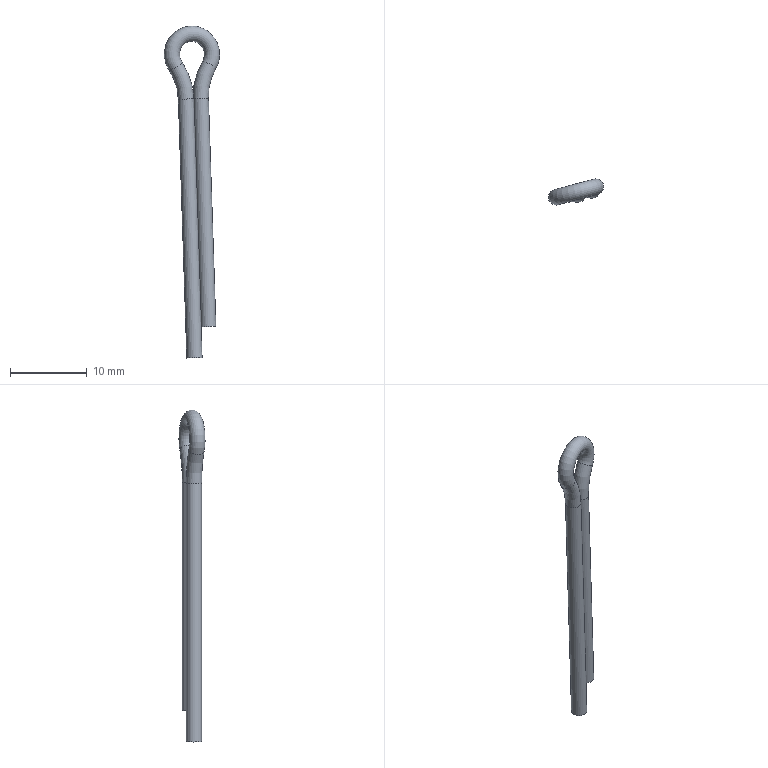Component | NX | 1 | 1 solid | 7 faces | box 7.22 x 3.4 x 43.24 mm | volume 264 mm3 | torus 3 | cylinder 2 | plane 2 | commonest cylinder face diameters 2 x2
STEP:
#1=CARTESIAN_POINT('',(0.,0.,0.));
#2=DIRECTION('',(0.,0.,1.));
#3=DIRECTION('',(1.,0.,0.));
#4=AXIS2_PLACEMENT_3D('',#1,#2,#3);
#5=CARTESIAN_POINT('',(-221.029,-44.318,113.398));
#6=VERTEX_POINT('',#5);
#7=CARTESIAN_POINT('',(-221.287,-43.352,113.39));
#8=DIRECTION('',(0.03267,-0.,-0.9995));
#9=DIRECTION('',(0.2584,-0.966,0.008448));
#10=AXIS2_PLACEMENT_3D('',#7,#8,#9);
#11=CIRCLE('',#10,1.);
#12=CARTESIAN_POINT('',(-221.287,-43.352,113.39));
#13=DIRECTION('',(0.03267,0.,-0.9995));
#14=DIRECTION('',(-0.2584,0.966,-0.008448));
#15=AXIS2_PLACEMENT_3D('',#12,#13,#14);
#16=CYLINDRICAL_SURFACE('',#15,1.);
#17=CARTESIAN_POINT('',(3.142,-0.));
#18=DIRECTION('',(1.,0.));
#19=VECTOR('',#18,1.);
#20=LINE('',#17,#19);
#21=(GEOMETRIC_REPRESENTATION_CONTEXT(2)PARAMETRIC_REPRESENTATION_CONTEXT()REPRESENTATION_CONTEXT('',''));
#22=DEFINITIONAL_REPRESENTATION('',(#20),#21);
#23=PCURVE('',#16,#22);
#24=CARTESIAN_POINT('',(-213.563,-41.284,113.642));
#25=DIRECTION('',(0.2584,-0.966,0.008448));
#26=DIRECTION('',(0.03267,-0.,-0.9995));
#27=AXIS2_PLACEMENT_3D('',#24,#25,#26);
#28=TOROIDAL_SURFACE('',#27,8.,1.);
#29=CARTESIAN_POINT('',(4.712,7.854));
#30=DIRECTION('',(0.,-1.));
#31=VECTOR('',#30,1.);
#32=LINE('',#29,#31);
#33=(GEOMETRIC_REPRESENTATION_CONTEXT(2)PARAMETRIC_REPRESENTATION_CONTEXT()REPRESENTATION_CONTEXT('',''));
#34=DEFINITIONAL_REPRESENTATION('',(#32),#33);
#35=PCURVE('',#28,#34);
#36=SURFACE_CURVE('',#11,(#23,#35),.PCURVE_S1.);
#37=EDGE_CURVE('',#6,#6,#36,.T.);
#38=ORIENTED_EDGE('',*,*,#37,.T.);
#39=CARTESIAN_POINT('',(-220.058,-44.318,83.701));
#40=VERTEX_POINT('',#39);
#41=CARTESIAN_POINT('',(-221.029,-44.318,113.398));
#42=CARTESIAN_POINT('',(-220.058,-44.318,83.701));
#43=B_SPLINE_CURVE_WITH_KNOTS('',1,(#41,#42),.UNSPECIFIED.,.F.,.F.,(2,2),(-0.,29.713),.PIECEWISE_BEZIER_KNOTS.);
#44=CARTESIAN_POINT('',(9.425,0.));
#45=DIRECTION('',(0.,1.));
#46=VECTOR('',#45,1.);
#47=LINE('',#44,#46);
#48=(GEOMETRIC_REPRESENTATION_CONTEXT(2)PARAMETRIC_REPRESENTATION_CONTEXT()REPRESENTATION_CONTEXT('',''));
#49=DEFINITIONAL_REPRESENTATION('',(#47),#48);
#50=PCURVE('',#16,#49);
#51=CARTESIAN_POINT('',(3.142,0.));
#52=DIRECTION('',(0.,1.));
#53=VECTOR('',#52,1.);
#54=LINE('',#51,#53);
#55=(GEOMETRIC_REPRESENTATION_CONTEXT(2)PARAMETRIC_REPRESENTATION_CONTEXT()REPRESENTATION_CONTEXT('',''));
#56=DEFINITIONAL_REPRESENTATION('',(#54),#55);
#57=PCURVE('',#16,#56);
#58=SEAM_CURVE('',#43,(#50,#57),.PCURVE_S1.);
#59=EDGE_CURVE('',#6,#40,#58,.T.);
#60=ORIENTED_EDGE('',*,*,#59,.T.);
#61=CARTESIAN_POINT('',(-220.316,-43.352,83.693));
#62=DIRECTION('',(0.03267,-0.,-0.9995));
#63=DIRECTION('',(0.2584,-0.966,0.008448));
#64=AXIS2_PLACEMENT_3D('',#61,#62,#63);
#65=CIRCLE('',#64,1.);
#66=CARTESIAN_POINT('',(3.142,29.713));
#67=DIRECTION('',(1.,0.));
#68=VECTOR('',#67,1.);
#69=LINE('',#66,#68);
#70=(GEOMETRIC_REPRESENTATION_CONTEXT(2)PARAMETRIC_REPRESENTATION_CONTEXT()REPRESENTATION_CONTEXT('',''));
#71=DEFINITIONAL_REPRESENTATION('',(#69),#70);
#72=PCURVE('',#16,#71);
#73=CARTESIAN_POINT('',(-220.316,-43.352,83.693));
#74=DIRECTION('',(0.03267,-0.,-0.9995));
#75=DIRECTION('',(0.2584,-0.966,0.008448));
#76=AXIS2_PLACEMENT_3D('',#73,#74,#75);
#77=PLANE('',#76);
#78=CARTESIAN_POINT('',(0.,0.));
#79=DIRECTION('',(1.,0.));
#80=AXIS2_PLACEMENT_2D('',#78,#79);
#81=CIRCLE('',#80,1.);
#82=(GEOMETRIC_REPRESENTATION_CONTEXT(2)PARAMETRIC_REPRESENTATION_CONTEXT()REPRESENTATION_CONTEXT('',''));
#83=DEFINITIONAL_REPRESENTATION('',(#81),#82);
#84=PCURVE('',#77,#83);
#85=SURFACE_CURVE('',#65,(#72,#84),.PCURVE_S1.);
#86=EDGE_CURVE('',#40,#40,#85,.T.);
#87=ORIENTED_EDGE('',*,*,#86,.F.);
#88=ORIENTED_EDGE('',*,*,#59,.F.);
#89=EDGE_LOOP('',(#38,#60,#87,#88));
#90=FACE_BOUND('',#89,.T.);
#91=ADVANCED_FACE('',(#90),#16,.T.);
#92=CARTESIAN_POINT('',(-219.943,-43.99,117.763));
#93=VERTEX_POINT('',#92);
#94=CARTESIAN_POINT('',(-220.201,-43.024,117.754));
#95=DIRECTION('',(-0.4947,-0.1398,-0.8577));
#96=DIRECTION('',(0.2584,-0.966,0.008448));
#97=AXIS2_PLACEMENT_3D('',#94,#95,#96);
#98=CIRCLE('',#97,1.);
#99=CARTESIAN_POINT('',(4.141,7.854));
#100=DIRECTION('',(0.,-1.));
#101=VECTOR('',#100,1.);
#102=LINE('',#99,#101);
#103=(GEOMETRIC_REPRESENTATION_CONTEXT(2)PARAMETRIC_REPRESENTATION_CONTEXT()REPRESENTATION_CONTEXT('',''));
#104=DEFINITIONAL_REPRESENTATION('',(#102),#103);
#105=PCURVE('',#28,#104);
#106=CARTESIAN_POINT('',(-222.442,-43.611,119.142));
#107=DIRECTION('',(-0.2584,0.966,-0.008448));
#108=DIRECTION('',(-0.03267,0.,0.9995));
#109=AXIS2_PLACEMENT_3D('',#106,#107,#108);
#110=TOROIDAL_SURFACE('',#109,2.7,1.);
#111=CARTESIAN_POINT('',(8.425,10.996));
#112=DIRECTION('',(0.,-1.));
#113=VECTOR('',#112,1.);
#114=LINE('',#111,#113);
#115=(GEOMETRIC_REPRESENTATION_CONTEXT(2)PARAMETRIC_REPRESENTATION_CONTEXT()REPRESENTATION_CONTEXT('',''));
#116=DEFINITIONAL_REPRESENTATION('',(#114),#115);
#117=PCURVE('',#110,#116);
#118=SURFACE_CURVE('',#98,(#105,#117),.PCURVE_S1.);
#119=EDGE_CURVE('',#93,#93,#118,.T.);
#120=ORIENTED_EDGE('',*,*,#119,.T.);
#121=CARTESIAN_POINT('',(-219.943,-43.99,117.763));
#122=CARTESIAN_POINT('',(-220.321,-44.097,117.108));
#123=CARTESIAN_POINT('',(-220.625,-44.184,116.409));
#124=CARTESIAN_POINT('',(-220.851,-44.251,115.679));
#125=CARTESIAN_POINT('',(-220.994,-44.296,114.926));
#126=CARTESIAN_POINT('',(-221.054,-44.318,114.162));
#127=CARTESIAN_POINT('',(-221.029,-44.318,113.398));
#128=(BOUNDED_CURVE()B_SPLINE_CURVE(6,(#121,#122,#123,#124,#125,#126,#127),.UNSPECIFIED.,.F.,.F.)B_SPLINE_CURVE_WITH_KNOTS((7,7),(4.141,4.712),.PIECEWISE_BEZIER_KNOTS.)CURVE()GEOMETRIC_REPRESENTATION_ITEM()RATIONAL_B_SPLINE_CURVE((1.004,1.001,0.9997,0.9992,0.9997,1.001,1.004))REPRESENTATION_ITEM(''));
#129=CARTESIAN_POINT('',(0.,1.571));
#130=DIRECTION('',(1.,0.));
#131=VECTOR('',#130,1.);
#132=LINE('',#129,#131);
#133=(GEOMETRIC_REPRESENTATION_CONTEXT(2)PARAMETRIC_REPRESENTATION_CONTEXT()REPRESENTATION_CONTEXT('',''));
#134=DEFINITIONAL_REPRESENTATION('',(#132),#133);
#135=PCURVE('',#28,#134);
#136=CARTESIAN_POINT('',(0.,7.854));
#137=DIRECTION('',(1.,0.));
#138=VECTOR('',#137,1.);
#139=LINE('',#136,#138);
#140=(GEOMETRIC_REPRESENTATION_CONTEXT(2)PARAMETRIC_REPRESENTATION_CONTEXT()REPRESENTATION_CONTEXT('',''));
#141=DEFINITIONAL_REPRESENTATION('',(#139),#140);
#142=PCURVE('',#28,#141);
#143=SEAM_CURVE('',#128,(#135,#142),.PCURVE_S1.);
#144=EDGE_CURVE('',#93,#6,#143,.T.);
#145=ORIENTED_EDGE('',*,*,#144,.T.);
#146=ORIENTED_EDGE('',*,*,#37,.F.);
#147=ORIENTED_EDGE('',*,*,#144,.F.);
#148=EDGE_LOOP('',(#120,#145,#146,#147));
#149=FACE_BOUND('',#148,.T.);
#150=ADVANCED_FACE('',(#149),#28,.T.);
#151=CARTESIAN_POINT('',(-224.328,-45.164,117.62));
#152=VERTEX_POINT('',#151);
#153=CARTESIAN_POINT('',(-224.587,-44.198,117.611));
#154=DIRECTION('',(-0.5497,-0.1398,0.8236));
#155=DIRECTION('',(0.2584,-0.966,0.008448));
#156=AXIS2_PLACEMENT_3D('',#153,#154,#155);
#157=CIRCLE('',#156,1.);
#158=CARTESIAN_POINT('',(4.141,10.996));
#159=DIRECTION('',(0.,-1.));
#160=VECTOR('',#159,1.);
#161=LINE('',#158,#160);
#162=(GEOMETRIC_REPRESENTATION_CONTEXT(2)PARAMETRIC_REPRESENTATION_CONTEXT()REPRESENTATION_CONTEXT('',''));
#163=DEFINITIONAL_REPRESENTATION('',(#161),#162);
#164=PCURVE('',#110,#163);
#165=CARTESIAN_POINT('',(-230.942,-45.938,113.074));
#166=DIRECTION('',(0.2584,-0.966,0.008448));
#167=DIRECTION('',(0.03267,-0.,-0.9995));
#168=AXIS2_PLACEMENT_3D('',#165,#166,#167);
#169=TOROIDAL_SURFACE('',#168,8.,1.);
#170=CARTESIAN_POINT('',(8.425,7.854));
#171=DIRECTION('',(0.,-1.));
#172=VECTOR('',#171,1.);
#173=LINE('',#170,#172);
#174=(GEOMETRIC_REPRESENTATION_CONTEXT(2)PARAMETRIC_REPRESENTATION_CONTEXT()REPRESENTATION_CONTEXT('',''));
#175=DEFINITIONAL_REPRESENTATION('',(#173),#174);
#176=PCURVE('',#169,#175);
#177=SURFACE_CURVE('',#157,(#164,#176),.PCURVE_S1.);
#178=EDGE_CURVE('',#152,#152,#177,.T.);
#179=ORIENTED_EDGE('',*,*,#178,.T.);
#180=CARTESIAN_POINT('',(-224.328,-45.164,117.62));
#181=CARTESIAN_POINT('',(-225.035,-45.344,118.678));
#182=CARTESIAN_POINT('',(-225.194,-45.374,120.127));
#183=CARTESIAN_POINT('',(-224.575,-45.195,121.618));
#184=CARTESIAN_POINT('',(-223.187,-44.815,122.641));
#185=CARTESIAN_POINT('',(-221.41,-44.339,122.699));
#186=CARTESIAN_POINT('',(-219.958,-43.959,121.769));
#187=CARTESIAN_POINT('',(-219.242,-43.78,120.322));
#188=CARTESIAN_POINT('',(-219.307,-43.81,118.865));
#189=CARTESIAN_POINT('',(-219.943,-43.99,117.763));
#190=B_SPLINE_CURVE_WITH_KNOTS('',9,(#180,#181,#182,#183,#184,#185,#186,#187,#188,#189),.UNSPECIFIED.,.F.,.F.,(10,10),(4.141,8.425),.PIECEWISE_BEZIER_KNOTS.);
#191=CARTESIAN_POINT('',(0.,4.712));
#192=DIRECTION('',(1.,0.));
#193=VECTOR('',#192,1.);
#194=LINE('',#191,#193);
#195=(GEOMETRIC_REPRESENTATION_CONTEXT(2)PARAMETRIC_REPRESENTATION_CONTEXT()REPRESENTATION_CONTEXT('',''));
#196=DEFINITIONAL_REPRESENTATION('',(#194),#195);
#197=PCURVE('',#110,#196);
#198=CARTESIAN_POINT('',(0.,10.996));
#199=DIRECTION('',(1.,0.));
#200=VECTOR('',#199,1.);
#201=LINE('',#198,#200);
#202=(GEOMETRIC_REPRESENTATION_CONTEXT(2)PARAMETRIC_REPRESENTATION_CONTEXT()REPRESENTATION_CONTEXT('',''));
#203=DEFINITIONAL_REPRESENTATION('',(#201),#202);
#204=PCURVE('',#110,#203);
#205=SEAM_CURVE('',#190,(#197,#204),.PCURVE_S1.);
#206=EDGE_CURVE('',#152,#93,#205,.T.);
#207=ORIENTED_EDGE('',*,*,#206,.T.);
#208=ORIENTED_EDGE('',*,*,#119,.F.);
#209=ORIENTED_EDGE('',*,*,#206,.F.);
#210=EDGE_LOOP('',(#179,#207,#208,#209));
#211=FACE_BOUND('',#210,.T.);
#212=ADVANCED_FACE('',(#211),#110,.T.);
#213=CARTESIAN_POINT('',(-222.96,-44.836,113.335));
#214=VERTEX_POINT('',#213);
#215=CARTESIAN_POINT('',(-223.218,-43.87,113.327));
#216=DIRECTION('',(-0.03267,0.,0.9995));
#217=DIRECTION('',(0.2584,-0.966,0.008448));
#218=AXIS2_PLACEMENT_3D('',#215,#216,#217);
#219=CIRCLE('',#218,1.);
#220=CARTESIAN_POINT('',(7.854,7.854));
#221=DIRECTION('',(0.,-1.));
#222=VECTOR('',#221,1.);
#223=LINE('',#220,#222);
#224=(GEOMETRIC_REPRESENTATION_CONTEXT(2)PARAMETRIC_REPRESENTATION_CONTEXT()REPRESENTATION_CONTEXT('',''));
#225=DEFINITIONAL_REPRESENTATION('',(#223),#224);
#226=PCURVE('',#169,#225);
#227=CARTESIAN_POINT('',(-223.218,-43.87,113.327));
#228=DIRECTION('',(0.03267,0.,-0.9995));
#229=DIRECTION('',(-0.2584,0.966,-0.008448));
#230=AXIS2_PLACEMENT_3D('',#227,#228,#229);
#231=CYLINDRICAL_SURFACE('',#230,1.);
#232=CARTESIAN_POINT('',(9.425,0.));
#233=DIRECTION('',(-1.,0.));
#234=VECTOR('',#233,1.);
#235=LINE('',#232,#234);
#236=(GEOMETRIC_REPRESENTATION_CONTEXT(2)PARAMETRIC_REPRESENTATION_CONTEXT()REPRESENTATION_CONTEXT('',''));
#237=DEFINITIONAL_REPRESENTATION('',(#235),#236);
#238=PCURVE('',#231,#237);
#239=SURFACE_CURVE('',#219,(#226,#238),.PCURVE_S1.);
#240=EDGE_CURVE('',#214,#214,#239,.T.);
#241=ORIENTED_EDGE('',*,*,#240,.T.);
#242=CARTESIAN_POINT('',(-222.96,-44.836,113.335));
#243=CARTESIAN_POINT('',(-222.985,-44.836,114.099));
#244=CARTESIAN_POINT('',(-223.094,-44.858,114.857));
#245=CARTESIAN_POINT('',(-223.286,-44.903,115.599));
#246=CARTESIAN_POINT('',(-223.559,-44.97,116.314));
#247=CARTESIAN_POINT('',(-223.908,-45.057,116.99));
#248=CARTESIAN_POINT('',(-224.328,-45.164,117.62));
#249=(BOUNDED_CURVE()B_SPLINE_CURVE(6,(#242,#243,#244,#245,#246,#247,#248),.UNSPECIFIED.,.F.,.F.)B_SPLINE_CURVE_WITH_KNOTS((7,7),(1.571,2.142),.PIECEWISE_BEZIER_KNOTS.)CURVE()GEOMETRIC_REPRESENTATION_ITEM()RATIONAL_B_SPLINE_CURVE((1.004,1.001,0.9997,0.9992,0.9997,1.001,1.004))REPRESENTATION_ITEM(''));
#250=CARTESIAN_POINT('',(6.283,1.571));
#251=DIRECTION('',(1.,0.));
#252=VECTOR('',#251,1.);
#253=LINE('',#250,#252);
#254=(GEOMETRIC_REPRESENTATION_CONTEXT(2)PARAMETRIC_REPRESENTATION_CONTEXT()REPRESENTATION_CONTEXT('',''));
#255=DEFINITIONAL_REPRESENTATION('',(#253),#254);
#256=PCURVE('',#169,#255);
#257=CARTESIAN_POINT('',(6.283,7.854));
#258=DIRECTION('',(1.,0.));
#259=VECTOR('',#258,1.);
#260=LINE('',#257,#259);
#261=(GEOMETRIC_REPRESENTATION_CONTEXT(2)PARAMETRIC_REPRESENTATION_CONTEXT()REPRESENTATION_CONTEXT('',''));
#262=DEFINITIONAL_REPRESENTATION('',(#260),#261);
#263=PCURVE('',#169,#262);
#264=SEAM_CURVE('',#249,(#256,#263),.PCURVE_S1.);
#265=EDGE_CURVE('',#214,#152,#264,.T.);
#266=ORIENTED_EDGE('',*,*,#265,.T.);
#267=ORIENTED_EDGE('',*,*,#178,.F.);
#268=ORIENTED_EDGE('',*,*,#265,.F.);
#269=EDGE_LOOP('',(#241,#266,#267,#268));
#270=FACE_BOUND('',#269,.T.);
#271=ADVANCED_FACE('',(#270),#169,.T.);
#272=ORIENTED_EDGE('',*,*,#240,.F.);
#273=CARTESIAN_POINT('',(-221.858,-44.836,79.64));
#274=VERTEX_POINT('',#273);
#275=CARTESIAN_POINT('',(-222.96,-44.836,113.335));
#276=CARTESIAN_POINT('',(-221.858,-44.836,79.64));
#277=B_SPLINE_CURVE_WITH_KNOTS('',1,(#275,#276),.UNSPECIFIED.,.F.,.F.,(2,2),(0.,33.713),.PIECEWISE_BEZIER_KNOTS.);
#278=CARTESIAN_POINT('',(9.425,0.));
#279=DIRECTION('',(0.,1.));
#280=VECTOR('',#279,1.);
#281=LINE('',#278,#280);
#282=(GEOMETRIC_REPRESENTATION_CONTEXT(2)PARAMETRIC_REPRESENTATION_CONTEXT()REPRESENTATION_CONTEXT('',''));
#283=DEFINITIONAL_REPRESENTATION('',(#281),#282);
#284=PCURVE('',#231,#283);
#285=CARTESIAN_POINT('',(3.142,0.));
#286=DIRECTION('',(0.,1.));
#287=VECTOR('',#286,1.);
#288=LINE('',#285,#287);
#289=(GEOMETRIC_REPRESENTATION_CONTEXT(2)PARAMETRIC_REPRESENTATION_CONTEXT()REPRESENTATION_CONTEXT('',''));
#290=DEFINITIONAL_REPRESENTATION('',(#288),#289);
#291=PCURVE('',#231,#290);
#292=SEAM_CURVE('',#277,(#284,#291),.PCURVE_S1.);
#293=EDGE_CURVE('',#214,#274,#292,.T.);
#294=ORIENTED_EDGE('',*,*,#293,.T.);
#295=CARTESIAN_POINT('',(-222.117,-43.87,79.632));
#296=DIRECTION('',(-0.03267,0.,0.9995));
#297=DIRECTION('',(0.2584,-0.966,0.008448));
#298=AXIS2_PLACEMENT_3D('',#295,#296,#297);
#299=CIRCLE('',#298,1.);
#300=CARTESIAN_POINT('',(9.425,33.713));
#301=DIRECTION('',(-1.,0.));
#302=VECTOR('',#301,1.);
#303=LINE('',#300,#302);
#304=(GEOMETRIC_REPRESENTATION_CONTEXT(2)PARAMETRIC_REPRESENTATION_CONTEXT()REPRESENTATION_CONTEXT('',''));
#305=DEFINITIONAL_REPRESENTATION('',(#303),#304);
#306=PCURVE('',#231,#305);
#307=CARTESIAN_POINT('',(-222.117,-43.87,79.632));
#308=DIRECTION('',(-0.03267,0.,0.9995));
#309=DIRECTION('',(0.2584,-0.966,0.008448));
#310=AXIS2_PLACEMENT_3D('',#307,#308,#309);
#311=PLANE('',#310);
#312=CARTESIAN_POINT('',(0.,0.));
#313=DIRECTION('',(1.,-0.));
#314=AXIS2_PLACEMENT_2D('',#312,#313);
#315=CIRCLE('',#314,1.);
#316=(GEOMETRIC_REPRESENTATION_CONTEXT(2)PARAMETRIC_REPRESENTATION_CONTEXT()REPRESENTATION_CONTEXT('',''));
#317=DEFINITIONAL_REPRESENTATION('',(#315),#316);
#318=PCURVE('',#311,#317);
#319=SURFACE_CURVE('',#299,(#306,#318),.PCURVE_S1.);
#320=EDGE_CURVE('',#274,#274,#319,.T.);
#321=ORIENTED_EDGE('',*,*,#320,.T.);
#322=ORIENTED_EDGE('',*,*,#293,.F.);
#323=EDGE_LOOP('',(#272,#294,#321,#322));
#324=FACE_BOUND('',#323,.T.);
#325=ADVANCED_FACE('',(#324),#231,.T.);
#326=ORIENTED_EDGE('',*,*,#86,.T.);
#327=EDGE_LOOP('',(#326));
#328=FACE_BOUND('',#327,.T.);
#329=ADVANCED_FACE('',(#328),#77,.T.);
#330=ORIENTED_EDGE('',*,*,#320,.F.);
#331=EDGE_LOOP('',(#330));
#332=FACE_BOUND('',#331,.T.);
#333=ADVANCED_FACE('',(#332),#311,.F.);
#334=CLOSED_SHELL('',(#91,#150,#212,#271,#325,#329,#333));
#335=MANIFOLD_SOLID_BREP('',#334);
#336=(LENGTH_UNIT()NAMED_UNIT(*)SI_UNIT(.MILLI.,.METRE.));
#337=UNCERTAINTY_MEASURE_WITH_UNIT(LENGTH_MEASURE(0.00001),#336,'','');
#338=(NAMED_UNIT(*)PLANE_ANGLE_UNIT()SI_UNIT($,.RADIAN.));
#339=(NAMED_UNIT(*)SI_UNIT($,.STERADIAN.)SOLID_ANGLE_UNIT());
#340=(GEOMETRIC_REPRESENTATION_CONTEXT(3)GLOBAL_UNCERTAINTY_ASSIGNED_CONTEXT((#337))GLOBAL_UNIT_ASSIGNED_CONTEXT((#336,#338,#339))REPRESENTATION_CONTEXT('',''));
#341=ADVANCED_BREP_SHAPE_REPRESENTATION('',(#4,#335),#340);